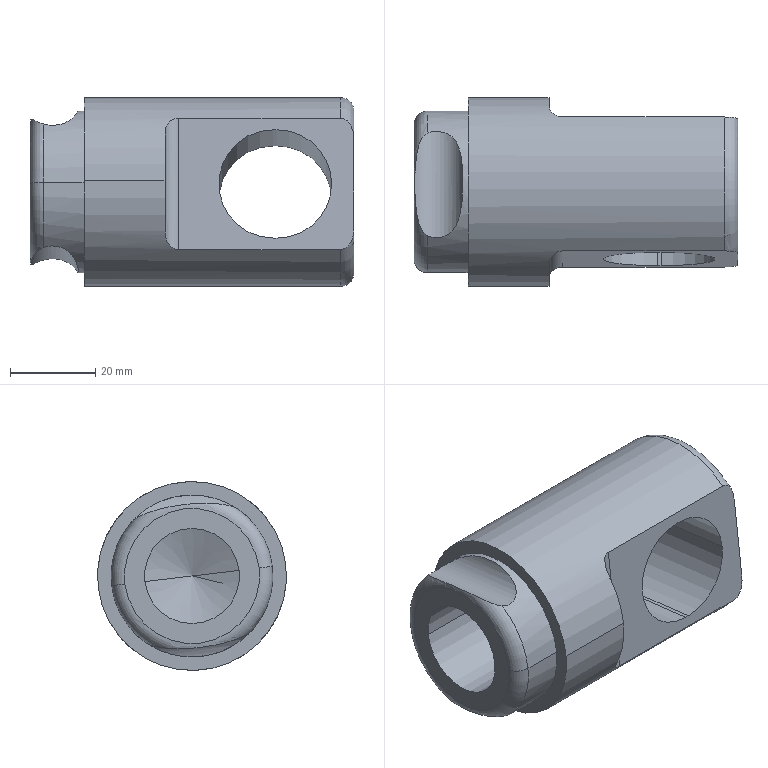Component | SolidWorks | DNR-71M20100BBEF2xx-A_504806-1_DNR-71M20100BBEF2xx-A_500780-1 | 1 solid | 28 faces | volume 71419 mm3 | cylinder 13 | plane 9 | torus 4 | cone 2 | commonest cylinder face diameters 25.654 x3 22.377 x2 44.45 x2 38.1 x2 12.7 x2 6.35 x2